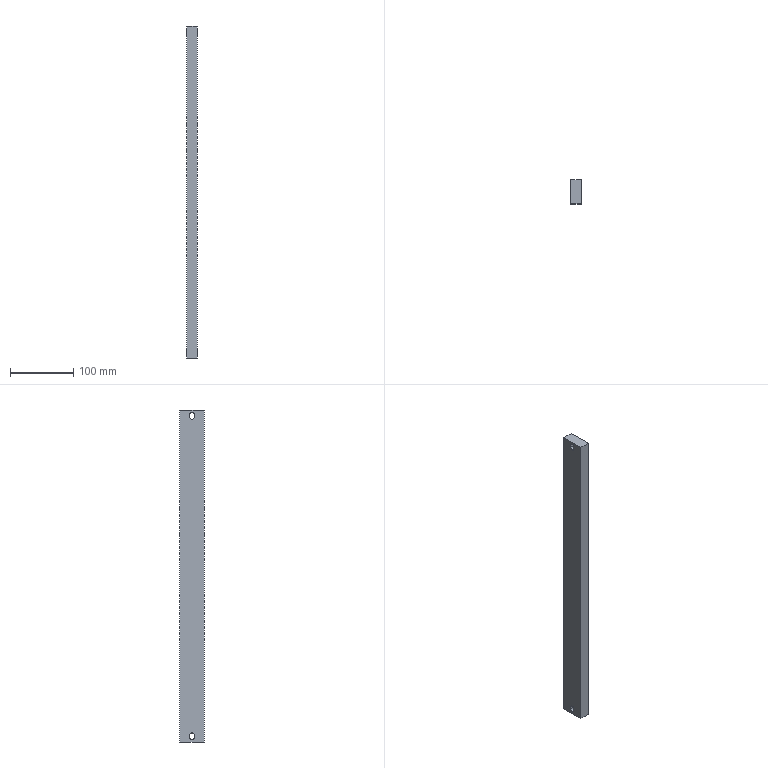Component | SolidWorks | NameDuplicate-1Crossbar-1 | 1 solid | 16 faces | box 16 x 38 x 523 mm | volume 315856 mm3 | plane 10 | cylinder 6 | commonest cylinder face diameters 7 x6
build123d program:
from build123d import *

# Parameters (mm, degrees)
SKETCH1_W           = 523
SKETCH1_H           = 38
BOSS_EXTRUDE1_DEPTH = 16


with BuildPart() as part:
    # Sketch1 → Boss-Extrude1 (new body)
    with BuildSketch(Plane.XY.offset(8)):
        Rectangle(SKETCH1_W, SKETCH1_H)
        with BuildLine():
            Line((-250.5, -3.5), (-254.5, -3.5))
            ThreePointArc((-254.5, -3.5), (-258, 0), (-254.5, 3.5))
            Line((-254.5, 3.5), (-250.5, 3.5))
            ThreePointArc((-250.5, 3.5), (-247, 0), (-250.5, -3.5))
        make_face(mode=Mode.SUBTRACT)
        with BuildLine():
            Line((254.5, -3.5), (250.5, -3.5))
            ThreePointArc((250.5, -3.5), (247, 0), (250.5, 3.5))
            Line((250.5, 3.5), (254.5, 3.5))
            ThreePointArc((254.5, 3.5), (258, 0), (254.5, -3.5))
        make_face(mode=Mode.SUBTRACT)
    extrude(amount=-BOSS_EXTRUDE1_DEPTH)


solid = part.part

# Placed as in the assembly
solid = solid.moved(Location((-405, 406, 0), (0, 90, 0)))
STEP:
#1=CARTESIAN_POINT('',(-15.63,15.984,10.157));
#2=VERTEX_POINT('',#1);
#3=CARTESIAN_POINT('',(-15.63,16.122,10.02));
#4=VERTEX_POINT('',#3);
#5=CARTESIAN_POINT('',(-15.63,15.984,10.02));
#6=DIRECTION('',(-1.,0.,0.));
#7=DIRECTION('',(0.,0.,-1.));
#8=AXIS2_PLACEMENT_3D('',#5,#6,#7);
#9=CIRCLE('',#8,0.1378);
#10=EDGE_CURVE('',#2,#4,#9,.T.);
#11=ORIENTED_EDGE('',*,*,#10,.F.);
#12=CARTESIAN_POINT('',(-16.26,15.984,10.157));
#13=VERTEX_POINT('',#12);
#14=CARTESIAN_POINT('',(-15.63,15.984,10.157));
#15=DIRECTION('',(-1.,0.,0.));
#16=VECTOR('',#15,39.37);
#17=LINE('',#14,#16);
#18=EDGE_CURVE('',#2,#13,#17,.T.);
#19=ORIENTED_EDGE('',*,*,#18,.T.);
#20=CARTESIAN_POINT('',(-16.26,16.122,10.02));
#21=VERTEX_POINT('',#20);
#22=CARTESIAN_POINT('',(-16.26,15.984,10.02));
#23=DIRECTION('',(-1.,0.,0.));
#24=DIRECTION('',(0.,0.,-1.));
#25=AXIS2_PLACEMENT_3D('',#22,#23,#24);
#26=CIRCLE('',#25,0.1378);
#27=EDGE_CURVE('',#13,#21,#26,.T.);
#28=ORIENTED_EDGE('',*,*,#27,.T.);
#29=CARTESIAN_POINT('',(-15.63,16.122,10.02));
#30=DIRECTION('',(-1.,0.,0.));
#31=VECTOR('',#30,39.37);
#32=LINE('',#29,#31);
#33=EDGE_CURVE('',#4,#21,#32,.T.);
#34=ORIENTED_EDGE('',*,*,#33,.F.);
#35=EDGE_LOOP('',(#11,#19,#28,#34));
#36=FACE_OUTER_BOUND('',#35,.T.);
#37=CARTESIAN_POINT('',(-15.63,15.984,10.02));
#38=DIRECTION('',(-1.,0.,0.));
#39=DIRECTION('',(0.,0.,1.));
#40=AXIS2_PLACEMENT_3D('',#37,#38,#39);
#41=CYLINDRICAL_SURFACE('',#40,0.1378);
#42=ADVANCED_FACE('',(#36),#41,.F.);
#43=CARTESIAN_POINT('',(-15.63,15.984,-9.724));
#44=VERTEX_POINT('',#43);
#45=CARTESIAN_POINT('',(-15.63,16.122,-9.862));
#46=VERTEX_POINT('',#45);
#47=CARTESIAN_POINT('',(-15.63,15.984,-9.862));
#48=DIRECTION('',(-1.,0.,0.));
#49=DIRECTION('',(0.,0.,-1.));
#50=AXIS2_PLACEMENT_3D('',#47,#48,#49);
#51=CIRCLE('',#50,0.1378);
#52=EDGE_CURVE('',#44,#46,#51,.T.);
#53=ORIENTED_EDGE('',*,*,#52,.F.);
#54=CARTESIAN_POINT('',(-16.26,15.984,-9.724));
#55=VERTEX_POINT('',#54);
#56=CARTESIAN_POINT('',(-15.63,15.984,-9.724));
#57=DIRECTION('',(-1.,0.,0.));
#58=VECTOR('',#57,39.37);
#59=LINE('',#56,#58);
#60=EDGE_CURVE('',#44,#55,#59,.T.);
#61=ORIENTED_EDGE('',*,*,#60,.T.);
#62=CARTESIAN_POINT('',(-16.26,16.122,-9.862));
#63=VERTEX_POINT('',#62);
#64=CARTESIAN_POINT('',(-16.26,15.984,-9.862));
#65=DIRECTION('',(-1.,0.,0.));
#66=DIRECTION('',(0.,0.,-1.));
#67=AXIS2_PLACEMENT_3D('',#64,#65,#66);
#68=CIRCLE('',#67,0.1378);
#69=EDGE_CURVE('',#55,#63,#68,.T.);
#70=ORIENTED_EDGE('',*,*,#69,.T.);
#71=CARTESIAN_POINT('',(-15.63,16.122,-9.862));
#72=DIRECTION('',(-1.,0.,0.));
#73=VECTOR('',#72,39.37);
#74=LINE('',#71,#73);
#75=EDGE_CURVE('',#46,#63,#74,.T.);
#76=ORIENTED_EDGE('',*,*,#75,.F.);
#77=EDGE_LOOP('',(#53,#61,#70,#76));
#78=FACE_OUTER_BOUND('',#77,.T.);
#79=CARTESIAN_POINT('',(-15.63,15.984,-9.862));
#80=DIRECTION('',(-1.,0.,0.));
#81=DIRECTION('',(0.,0.,1.));
#82=AXIS2_PLACEMENT_3D('',#79,#80,#81);
#83=CYLINDRICAL_SURFACE('',#82,0.1378);
#84=ADVANCED_FACE('',(#78),#83,.F.);
#85=CARTESIAN_POINT('',(-16.26,15.236,-10.295));
#86=VERTEX_POINT('',#85);
#87=CARTESIAN_POINT('',(-16.26,15.236,10.295));
#88=VERTEX_POINT('',#87);
#89=CARTESIAN_POINT('',(-16.26,15.236,-10.295));
#90=DIRECTION('',(0.,0.,1.));
#91=VECTOR('',#90,39.37);
#92=LINE('',#89,#91);
#93=EDGE_CURVE('',#86,#88,#92,.T.);
#94=ORIENTED_EDGE('',*,*,#93,.F.);
#95=CARTESIAN_POINT('',(-15.63,15.236,-10.295));
#96=VERTEX_POINT('',#95);
#97=CARTESIAN_POINT('',(-15.63,15.236,-10.295));
#98=DIRECTION('',(-1.,0.,0.));
#99=VECTOR('',#98,39.37);
#100=LINE('',#97,#99);
#101=EDGE_CURVE('',#96,#86,#100,.T.);
#102=ORIENTED_EDGE('',*,*,#101,.F.);
#103=CARTESIAN_POINT('',(-15.63,15.236,10.295));
#104=VERTEX_POINT('',#103);
#105=CARTESIAN_POINT('',(-15.63,15.236,-10.295));
#106=DIRECTION('',(0.,0.,1.));
#107=VECTOR('',#106,39.37);
#108=LINE('',#105,#107);
#109=EDGE_CURVE('',#96,#104,#108,.T.);
#110=ORIENTED_EDGE('',*,*,#109,.T.);
#111=CARTESIAN_POINT('',(-15.63,15.236,10.295));
#112=DIRECTION('',(-1.,0.,0.));
#113=VECTOR('',#112,39.37);
#114=LINE('',#111,#113);
#115=EDGE_CURVE('',#104,#88,#114,.T.);
#116=ORIENTED_EDGE('',*,*,#115,.T.);
#117=EDGE_LOOP('',(#94,#102,#110,#116));
#118=FACE_OUTER_BOUND('',#117,.T.);
#119=CARTESIAN_POINT('',(-15.63,15.236,-10.295));
#120=DIRECTION('',(-0.,-1.,0.));
#121=DIRECTION('',(1.,-0.,-0.));
#122=AXIS2_PLACEMENT_3D('',#119,#120,#121);
#123=PLANE('',#122);
#124=ADVANCED_FACE('',(#118),#123,.T.);
#125=CARTESIAN_POINT('',(-16.26,16.732,-10.295));
#126=VERTEX_POINT('',#125);
#127=CARTESIAN_POINT('',(-16.26,16.732,-10.295));
#128=DIRECTION('',(-0.,-1.,0.));
#129=VECTOR('',#128,39.37);
#130=LINE('',#127,#129);
#131=EDGE_CURVE('',#126,#86,#130,.T.);
#132=ORIENTED_EDGE('',*,*,#131,.F.);
#133=CARTESIAN_POINT('',(-15.63,16.732,-10.295));
#134=VERTEX_POINT('',#133);
#135=CARTESIAN_POINT('',(-15.63,16.732,-10.295));
#136=DIRECTION('',(-1.,0.,0.));
#137=VECTOR('',#136,39.37);
#138=LINE('',#135,#137);
#139=EDGE_CURVE('',#134,#126,#138,.T.);
#140=ORIENTED_EDGE('',*,*,#139,.F.);
#141=CARTESIAN_POINT('',(-15.63,16.732,-10.295));
#142=DIRECTION('',(-0.,-1.,0.));
#143=VECTOR('',#142,39.37);
#144=LINE('',#141,#143);
#145=EDGE_CURVE('',#134,#96,#144,.T.);
#146=ORIENTED_EDGE('',*,*,#145,.T.);
#147=ORIENTED_EDGE('',*,*,#101,.T.);
#148=EDGE_LOOP('',(#132,#140,#146,#147));
#149=FACE_OUTER_BOUND('',#148,.T.);
#150=CARTESIAN_POINT('',(-15.63,16.732,-10.295));
#151=DIRECTION('',(-0.,-0.,-1.));
#152=DIRECTION('',(-1.,0.,0.));
#153=AXIS2_PLACEMENT_3D('',#150,#151,#152);
#154=PLANE('',#153);
#155=ADVANCED_FACE('',(#149),#154,.T.);
#156=CARTESIAN_POINT('',(-16.26,16.732,10.295));
#157=VERTEX_POINT('',#156);
#158=CARTESIAN_POINT('',(-16.26,16.732,10.295));
#159=DIRECTION('',(-0.,-0.,-1.));
#160=VECTOR('',#159,39.37);
#161=LINE('',#158,#160);
#162=EDGE_CURVE('',#157,#126,#161,.T.);
#163=ORIENTED_EDGE('',*,*,#162,.F.);
#164=CARTESIAN_POINT('',(-15.63,16.732,10.295));
#165=VERTEX_POINT('',#164);
#166=CARTESIAN_POINT('',(-15.63,16.732,10.295));
#167=DIRECTION('',(-1.,0.,0.));
#168=VECTOR('',#167,39.37);
#169=LINE('',#166,#168);
#170=EDGE_CURVE('',#165,#157,#169,.T.);
#171=ORIENTED_EDGE('',*,*,#170,.F.);
#172=CARTESIAN_POINT('',(-15.63,16.732,10.295));
#173=DIRECTION('',(-0.,-0.,-1.));
#174=VECTOR('',#173,39.37);
#175=LINE('',#172,#174);
#176=EDGE_CURVE('',#165,#134,#175,.T.);
#177=ORIENTED_EDGE('',*,*,#176,.T.);
#178=ORIENTED_EDGE('',*,*,#139,.T.);
#179=EDGE_LOOP('',(#163,#171,#177,#178));
#180=FACE_OUTER_BOUND('',#179,.T.);
#181=CARTESIAN_POINT('',(-15.63,16.732,10.295));
#182=DIRECTION('',(0.,1.,-0.));
#183=DIRECTION('',(-0.,-0.,-1.));
#184=AXIS2_PLACEMENT_3D('',#181,#182,#183);
#185=PLANE('',#184);
#186=ADVANCED_FACE('',(#180),#185,.T.);
#187=CARTESIAN_POINT('',(-16.26,15.236,10.295));
#188=DIRECTION('',(0.,1.,-0.));
#189=VECTOR('',#188,39.37);
#190=LINE('',#187,#189);
#191=EDGE_CURVE('',#88,#157,#190,.T.);
#192=ORIENTED_EDGE('',*,*,#191,.F.);
#193=ORIENTED_EDGE('',*,*,#115,.F.);
#194=CARTESIAN_POINT('',(-15.63,15.236,10.295));
#195=DIRECTION('',(0.,1.,-0.));
#196=VECTOR('',#195,39.37);
#197=LINE('',#194,#196);
#198=EDGE_CURVE('',#104,#165,#197,.T.);
#199=ORIENTED_EDGE('',*,*,#198,.T.);
#200=ORIENTED_EDGE('',*,*,#170,.T.);
#201=EDGE_LOOP('',(#192,#193,#199,#200));
#202=FACE_OUTER_BOUND('',#201,.T.);
#203=CARTESIAN_POINT('',(-15.63,15.236,10.295));
#204=DIRECTION('',(0.,0.,1.));
#205=DIRECTION('',(1.,-0.,-0.));
#206=AXIS2_PLACEMENT_3D('',#203,#204,#205);
#207=PLANE('',#206);
#208=ADVANCED_FACE('',(#202),#207,.T.);
#209=CARTESIAN_POINT('',(-15.63,15.846,9.862));
#210=VERTEX_POINT('',#209);
#211=CARTESIAN_POINT('',(-15.63,15.846,10.02));
#212=VERTEX_POINT('',#211);
#213=CARTESIAN_POINT('',(-15.63,15.846,10.02));
#214=DIRECTION('',(0.,0.,1.));
#215=VECTOR('',#214,39.37);
#216=LINE('',#213,#215);
#217=EDGE_CURVE('',#210,#212,#216,.T.);
#218=ORIENTED_EDGE('',*,*,#217,.T.);
#219=CARTESIAN_POINT('',(-15.63,15.984,10.02));
#220=DIRECTION('',(-1.,0.,0.));
#221=DIRECTION('',(0.,0.,-1.));
#222=AXIS2_PLACEMENT_3D('',#219,#220,#221);
#223=CIRCLE('',#222,0.1378);
#224=EDGE_CURVE('',#212,#2,#223,.T.);
#225=ORIENTED_EDGE('',*,*,#224,.T.);
#226=ORIENTED_EDGE('',*,*,#10,.T.);
#227=CARTESIAN_POINT('',(-15.63,16.122,9.862));
#228=VERTEX_POINT('',#227);
#229=CARTESIAN_POINT('',(-15.63,16.122,9.862));
#230=DIRECTION('',(-0.,-0.,-1.));
#231=VECTOR('',#230,39.37);
#232=LINE('',#229,#231);
#233=EDGE_CURVE('',#4,#228,#232,.T.);
#234=ORIENTED_EDGE('',*,*,#233,.T.);
#235=CARTESIAN_POINT('',(-15.63,15.984,9.862));
#236=DIRECTION('',(-1.,0.,0.));
#237=DIRECTION('',(0.,0.,-1.));
#238=AXIS2_PLACEMENT_3D('',#235,#236,#237);
#239=CIRCLE('',#238,0.1378);
#240=EDGE_CURVE('',#228,#210,#239,.T.);
#241=ORIENTED_EDGE('',*,*,#240,.T.);
#242=EDGE_LOOP('',(#218,#225,#226,#234,#241));
#243=FACE_BOUND('',#242,.T.);
#244=CARTESIAN_POINT('',(-15.63,15.846,-10.02));
#245=VERTEX_POINT('',#244);
#246=CARTESIAN_POINT('',(-15.63,15.846,-9.862));
#247=VERTEX_POINT('',#246);
#248=CARTESIAN_POINT('',(-15.63,15.846,-9.862));
#249=DIRECTION('',(0.,0.,1.));
#250=VECTOR('',#249,39.37);
#251=LINE('',#248,#250);
#252=EDGE_CURVE('',#245,#247,#251,.T.);
#253=ORIENTED_EDGE('',*,*,#252,.T.);
#254=CARTESIAN_POINT('',(-15.63,15.984,-9.862));
#255=DIRECTION('',(-1.,0.,0.));
#256=DIRECTION('',(0.,0.,-1.));
#257=AXIS2_PLACEMENT_3D('',#254,#255,#256);
#258=CIRCLE('',#257,0.1378);
#259=EDGE_CURVE('',#247,#44,#258,.T.);
#260=ORIENTED_EDGE('',*,*,#259,.T.);
#261=ORIENTED_EDGE('',*,*,#52,.T.);
#262=CARTESIAN_POINT('',(-15.63,16.122,-10.02));
#263=VERTEX_POINT('',#262);
#264=CARTESIAN_POINT('',(-15.63,16.122,-10.02));
#265=DIRECTION('',(-0.,-0.,-1.));
#266=VECTOR('',#265,39.37);
#267=LINE('',#264,#266);
#268=EDGE_CURVE('',#46,#263,#267,.T.);
#269=ORIENTED_EDGE('',*,*,#268,.T.);
#270=CARTESIAN_POINT('',(-15.63,15.984,-10.02));
#271=DIRECTION('',(-1.,0.,0.));
#272=DIRECTION('',(0.,0.,-1.));
#273=AXIS2_PLACEMENT_3D('',#270,#271,#272);
#274=CIRCLE('',#273,0.1378);
#275=EDGE_CURVE('',#263,#245,#274,.T.);
#276=ORIENTED_EDGE('',*,*,#275,.T.);
#277=EDGE_LOOP('',(#253,#260,#261,#269,#276));
#278=FACE_BOUND('',#277,.T.);
#279=ORIENTED_EDGE('',*,*,#109,.F.);
#280=ORIENTED_EDGE('',*,*,#145,.F.);
#281=ORIENTED_EDGE('',*,*,#176,.F.);
#282=ORIENTED_EDGE('',*,*,#198,.F.);
#283=EDGE_LOOP('',(#279,#280,#281,#282));
#284=FACE_OUTER_BOUND('',#283,.T.);
#285=CARTESIAN_POINT('',(-15.63,15.984,-0.));
#286=DIRECTION('',(-1.,0.,0.));
#287=DIRECTION('',(0.,0.,1.));
#288=AXIS2_PLACEMENT_3D('',#285,#286,#287);
#289=PLANE('',#288);
#290=ADVANCED_FACE('',(#243,#278,#284),#289,.F.);
#291=CARTESIAN_POINT('',(-16.26,15.846,10.02));
#292=VERTEX_POINT('',#291);
#293=CARTESIAN_POINT('',(-16.26,15.984,10.02));
#294=DIRECTION('',(-1.,0.,0.));
#295=DIRECTION('',(0.,0.,-1.));
#296=AXIS2_PLACEMENT_3D('',#293,#294,#295);
#297=CIRCLE('',#296,0.1378);
#298=EDGE_CURVE('',#292,#13,#297,.T.);
#299=ORIENTED_EDGE('',*,*,#298,.F.);
#300=CARTESIAN_POINT('',(-16.26,15.846,9.862));
#301=VERTEX_POINT('',#300);
#302=CARTESIAN_POINT('',(-16.26,15.846,10.02));
#303=DIRECTION('',(0.,0.,1.));
#304=VECTOR('',#303,39.37);
#305=LINE('',#302,#304);
#306=EDGE_CURVE('',#301,#292,#305,.T.);
#307=ORIENTED_EDGE('',*,*,#306,.F.);
#308=CARTESIAN_POINT('',(-16.26,16.122,9.862));
#309=VERTEX_POINT('',#308);
#310=CARTESIAN_POINT('',(-16.26,15.984,9.862));
#311=DIRECTION('',(-1.,0.,0.));
#312=DIRECTION('',(0.,0.,-1.));
#313=AXIS2_PLACEMENT_3D('',#310,#311,#312);
#314=CIRCLE('',#313,0.1378);
#315=EDGE_CURVE('',#309,#301,#314,.T.);
#316=ORIENTED_EDGE('',*,*,#315,.F.);
#317=CARTESIAN_POINT('',(-16.26,16.122,9.862));
#318=DIRECTION('',(-0.,-0.,-1.));
#319=VECTOR('',#318,39.37);
#320=LINE('',#317,#319);
#321=EDGE_CURVE('',#21,#309,#320,.T.);
#322=ORIENTED_EDGE('',*,*,#321,.F.);
#323=ORIENTED_EDGE('',*,*,#27,.F.);
#324=EDGE_LOOP('',(#299,#307,#316,#322,#323));
#325=FACE_BOUND('',#324,.T.);
#326=CARTESIAN_POINT('',(-16.26,15.846,-9.862));
#327=VERTEX_POINT('',#326);
#328=CARTESIAN_POINT('',(-16.26,15.984,-9.862));
#329=DIRECTION('',(-1.,0.,0.));
#330=DIRECTION('',(0.,0.,-1.));
#331=AXIS2_PLACEMENT_3D('',#328,#329,#330);
#332=CIRCLE('',#331,0.1378);
#333=EDGE_CURVE('',#327,#55,#332,.T.);
#334=ORIENTED_EDGE('',*,*,#333,.F.);
#335=CARTESIAN_POINT('',(-16.26,15.846,-10.02));
#336=VERTEX_POINT('',#335);
#337=CARTESIAN_POINT('',(-16.26,15.846,-9.862));
#338=DIRECTION('',(0.,0.,1.));
#339=VECTOR('',#338,39.37);
#340=LINE('',#337,#339);
#341=EDGE_CURVE('',#336,#327,#340,.T.);
#342=ORIENTED_EDGE('',*,*,#341,.F.);
#343=CARTESIAN_POINT('',(-16.26,16.122,-10.02));
#344=VERTEX_POINT('',#343);
#345=CARTESIAN_POINT('',(-16.26,15.984,-10.02));
#346=DIRECTION('',(-1.,0.,0.));
#347=DIRECTION('',(0.,0.,-1.));
#348=AXIS2_PLACEMENT_3D('',#345,#346,#347);
#349=CIRCLE('',#348,0.1378);
#350=EDGE_CURVE('',#344,#336,#349,.T.);
#351=ORIENTED_EDGE('',*,*,#350,.F.);
#352=CARTESIAN_POINT('',(-16.26,16.122,-10.02));
#353=DIRECTION('',(-0.,-0.,-1.));
#354=VECTOR('',#353,39.37);
#355=LINE('',#352,#354);
#356=EDGE_CURVE('',#63,#344,#355,.T.);
#357=ORIENTED_EDGE('',*,*,#356,.F.);
#358=ORIENTED_EDGE('',*,*,#69,.F.);
#359=EDGE_LOOP('',(#334,#342,#351,#357,#358));
#360=FACE_BOUND('',#359,.T.);
#361=ORIENTED_EDGE('',*,*,#93,.T.);
#362=ORIENTED_EDGE('',*,*,#191,.T.);
#363=ORIENTED_EDGE('',*,*,#162,.T.);
#364=ORIENTED_EDGE('',*,*,#131,.T.);
#365=EDGE_LOOP('',(#361,#362,#363,#364));
#366=FACE_OUTER_BOUND('',#365,.T.);
#367=CARTESIAN_POINT('',(-16.26,15.984,-0.));
#368=DIRECTION('',(-1.,0.,0.));
#369=DIRECTION('',(0.,0.,1.));
#370=AXIS2_PLACEMENT_3D('',#367,#368,#369);
#371=PLANE('',#370);
#372=ADVANCED_FACE('',(#325,#360,#366),#371,.T.);
#373=ORIENTED_EDGE('',*,*,#60,.F.);
#374=ORIENTED_EDGE('',*,*,#259,.F.);
#375=CARTESIAN_POINT('',(-15.63,15.846,-9.862));
#376=DIRECTION('',(-1.,0.,0.));
#377=VECTOR('',#376,39.37);
#378=LINE('',#375,#377);
#379=EDGE_CURVE('',#247,#327,#378,.T.);
#380=ORIENTED_EDGE('',*,*,#379,.T.);
#381=ORIENTED_EDGE('',*,*,#333,.T.);
#382=EDGE_LOOP('',(#373,#374,#380,#381));
#383=FACE_OUTER_BOUND('',#382,.T.);
#384=CARTESIAN_POINT('',(-15.63,15.984,-9.862));
#385=DIRECTION('',(-1.,0.,0.));
#386=DIRECTION('',(0.,0.,1.));
#387=AXIS2_PLACEMENT_3D('',#384,#385,#386);
#388=CYLINDRICAL_SURFACE('',#387,0.1378);
#389=ADVANCED_FACE('',(#383),#388,.F.);
#390=ORIENTED_EDGE('',*,*,#341,.T.);
#391=ORIENTED_EDGE('',*,*,#379,.F.);
#392=ORIENTED_EDGE('',*,*,#252,.F.);
#393=CARTESIAN_POINT('',(-15.63,15.846,-10.02));
#394=DIRECTION('',(-1.,0.,0.));
#395=VECTOR('',#394,39.37);
#396=LINE('',#393,#395);
#397=EDGE_CURVE('',#245,#336,#396,.T.);
#398=ORIENTED_EDGE('',*,*,#397,.T.);
#399=EDGE_LOOP('',(#390,#391,#392,#398));
#400=FACE_OUTER_BOUND('',#399,.T.);
#401=CARTESIAN_POINT('',(-15.63,15.846,-9.862));
#402=DIRECTION('',(-0.,-1.,0.));
#403=DIRECTION('',(0.,0.,1.));
#404=AXIS2_PLACEMENT_3D('',#401,#402,#403);
#405=PLANE('',#404);
#406=ADVANCED_FACE('',(#400),#405,.F.);
#407=ORIENTED_EDGE('',*,*,#350,.T.);
#408=ORIENTED_EDGE('',*,*,#397,.F.);
#409=ORIENTED_EDGE('',*,*,#275,.F.);
#410=CARTESIAN_POINT('',(-15.63,16.122,-10.02));
#411=DIRECTION('',(-1.,0.,0.));
#412=VECTOR('',#411,39.37);
#413=LINE('',#410,#412);
#414=EDGE_CURVE('',#263,#344,#413,.T.);
#415=ORIENTED_EDGE('',*,*,#414,.T.);
#416=EDGE_LOOP('',(#407,#408,#409,#415));
#417=FACE_OUTER_BOUND('',#416,.T.);
#418=CARTESIAN_POINT('',(-15.63,15.984,-10.02));
#419=DIRECTION('',(-1.,0.,0.));
#420=DIRECTION('',(0.,0.,1.));
#421=AXIS2_PLACEMENT_3D('',#418,#419,#420);
#422=CYLINDRICAL_SURFACE('',#421,0.1378);
#423=ADVANCED_FACE('',(#417),#422,.F.);
#424=ORIENTED_EDGE('',*,*,#356,.T.);
#425=ORIENTED_EDGE('',*,*,#414,.F.);
#426=ORIENTED_EDGE('',*,*,#268,.F.);
#427=ORIENTED_EDGE('',*,*,#75,.T.);
#428=EDGE_LOOP('',(#424,#425,#426,#427));
#429=FACE_OUTER_BOUND('',#428,.T.);
#430=CARTESIAN_POINT('',(-15.63,16.122,-10.02));
#431=DIRECTION('',(0.,1.,-0.));
#432=DIRECTION('',(-0.,-0.,-1.));
#433=AXIS2_PLACEMENT_3D('',#430,#431,#432);
#434=PLANE('',#433);
#435=ADVANCED_FACE('',(#429),#434,.F.);
#436=ORIENTED_EDGE('',*,*,#18,.F.);
#437=ORIENTED_EDGE('',*,*,#224,.F.);
#438=CARTESIAN_POINT('',(-15.63,15.846,10.02));
#439=DIRECTION('',(-1.,0.,0.));
#440=VECTOR('',#439,39.37);
#441=LINE('',#438,#440);
#442=EDGE_CURVE('',#212,#292,#441,.T.);
#443=ORIENTED_EDGE('',*,*,#442,.T.);
#444=ORIENTED_EDGE('',*,*,#298,.T.);
#445=EDGE_LOOP('',(#436,#437,#443,#444));
#446=FACE_OUTER_BOUND('',#445,.T.);
#447=CARTESIAN_POINT('',(-15.63,15.984,10.02));
#448=DIRECTION('',(-1.,0.,0.));
#449=DIRECTION('',(0.,0.,1.));
#450=AXIS2_PLACEMENT_3D('',#447,#448,#449);
#451=CYLINDRICAL_SURFACE('',#450,0.1378);
#452=ADVANCED_FACE('',(#446),#451,.F.);
#453=ORIENTED_EDGE('',*,*,#306,.T.);
#454=ORIENTED_EDGE('',*,*,#442,.F.);
#455=ORIENTED_EDGE('',*,*,#217,.F.);
#456=CARTESIAN_POINT('',(-15.63,15.846,9.862));
#457=DIRECTION('',(-1.,0.,0.));
#458=VECTOR('',#457,39.37);
#459=LINE('',#456,#458);
#460=EDGE_CURVE('',#210,#301,#459,.T.);
#461=ORIENTED_EDGE('',*,*,#460,.T.);
#462=EDGE_LOOP('',(#453,#454,#455,#461));
#463=FACE_OUTER_BOUND('',#462,.T.);
#464=CARTESIAN_POINT('',(-15.63,15.846,10.02));
#465=DIRECTION('',(-0.,-1.,0.));
#466=DIRECTION('',(0.,0.,1.));
#467=AXIS2_PLACEMENT_3D('',#464,#465,#466);
#468=PLANE('',#467);
#469=ADVANCED_FACE('',(#463),#468,.F.);
#470=ORIENTED_EDGE('',*,*,#315,.T.);
#471=ORIENTED_EDGE('',*,*,#460,.F.);
#472=ORIENTED_EDGE('',*,*,#240,.F.);
#473=CARTESIAN_POINT('',(-15.63,16.122,9.862));
#474=DIRECTION('',(-1.,0.,0.));
#475=VECTOR('',#474,39.37);
#476=LINE('',#473,#475);
#477=EDGE_CURVE('',#228,#309,#476,.T.);
#478=ORIENTED_EDGE('',*,*,#477,.T.);
#479=EDGE_LOOP('',(#470,#471,#472,#478));
#480=FACE_OUTER_BOUND('',#479,.T.);
#481=CARTESIAN_POINT('',(-15.63,15.984,9.862));
#482=DIRECTION('',(-1.,0.,0.));
#483=DIRECTION('',(0.,0.,1.));
#484=AXIS2_PLACEMENT_3D('',#481,#482,#483);
#485=CYLINDRICAL_SURFACE('',#484,0.1378);
#486=ADVANCED_FACE('',(#480),#485,.F.);
#487=ORIENTED_EDGE('',*,*,#321,.T.);
#488=ORIENTED_EDGE('',*,*,#477,.F.);
#489=ORIENTED_EDGE('',*,*,#233,.F.);
#490=ORIENTED_EDGE('',*,*,#33,.T.);
#491=EDGE_LOOP('',(#487,#488,#489,#490));
#492=FACE_OUTER_BOUND('',#491,.T.);
#493=CARTESIAN_POINT('',(-15.63,16.122,9.862));
#494=DIRECTION('',(0.,1.,-0.));
#495=DIRECTION('',(-0.,-0.,-1.));
#496=AXIS2_PLACEMENT_3D('',#493,#494,#495);
#497=PLANE('',#496);
#498=ADVANCED_FACE('',(#492),#497,.F.);
#499=CLOSED_SHELL('',(#42,#84,#124,#155,#186,#208,#290,#372,#389,#406,#423,#435,#452,#469,#486,#498));
#500=MANIFOLD_SOLID_BREP('',#499);
#501=CARTESIAN_POINT('',(0.,0.,0.));
#502=DIRECTION('',(0.,0.,1.));
#503=DIRECTION('',(1.,0.,0.));
#504=AXIS2_PLACEMENT_3D('',#501,#502,#503);
#505=(LENGTH_UNIT()NAMED_UNIT(*)SI_UNIT($,.METRE.));
#506=LENGTH_MEASURE_WITH_UNIT(LENGTH_MEASURE(0.0254),#505);
#507=DIMENSIONAL_EXPONENTS(1.,0.,0.,0.,0.,0.,0.);
#508=(CONVERSION_BASED_UNIT('',#506)LENGTH_UNIT()NAMED_UNIT(#507));
#509=UNCERTAINTY_MEASURE_WITH_UNIT(LENGTH_MEASURE(0.00001),#508,'','');
#510=(NAMED_UNIT(*)PLANE_ANGLE_UNIT()SI_UNIT($,.RADIAN.));
#511=(NAMED_UNIT(*)SI_UNIT($,.STERADIAN.)SOLID_ANGLE_UNIT());
#512=(GEOMETRIC_REPRESENTATION_CONTEXT(3)GLOBAL_UNCERTAINTY_ASSIGNED_CONTEXT((#509))GLOBAL_UNIT_ASSIGNED_CONTEXT((#508,#510,#511))REPRESENTATION_CONTEXT('',''));
#513=ADVANCED_BREP_SHAPE_REPRESENTATION('',(#500,#504),#512);
#514=COLOUR_RGB('',0.7922,0.8196,0.9333);
#515=FILL_AREA_STYLE_COLOUR('',#514);
#516=FILL_AREA_STYLE('',(#515));
#517=SURFACE_STYLE_FILL_AREA(#516);
#518=SURFACE_SIDE_STYLE('',(#517));
#519=SURFACE_STYLE_USAGE(.BOTH.,#518);
#520=PRESENTATION_STYLE_ASSIGNMENT((#519));
#521=STYLED_ITEM('',(#520),#500);
#522=PRESENTATION_LAYER_ASSIGNMENT('','',(#521));
#523=(LENGTH_UNIT()NAMED_UNIT(*)SI_UNIT($,.METRE.));
#524=LENGTH_MEASURE_WITH_UNIT(LENGTH_MEASURE(0.0254),#523);
#525=DIMENSIONAL_EXPONENTS(1.,0.,0.,0.,0.,0.,0.);
#526=(CONVERSION_BASED_UNIT('',#524)LENGTH_UNIT()NAMED_UNIT(#525));
#527=UNCERTAINTY_MEASURE_WITH_UNIT(LENGTH_MEASURE(0.00001),#526,'','');
#528=(NAMED_UNIT(*)PLANE_ANGLE_UNIT()SI_UNIT($,.RADIAN.));
#529=(NAMED_UNIT(*)SI_UNIT($,.STERADIAN.)SOLID_ANGLE_UNIT());
#530=(GEOMETRIC_REPRESENTATION_CONTEXT(3)GLOBAL_UNCERTAINTY_ASSIGNED_CONTEXT((#527))GLOBAL_UNIT_ASSIGNED_CONTEXT((#526,#528,#529))REPRESENTATION_CONTEXT('',''));
#531=MECHANICAL_DESIGN_GEOMETRIC_PRESENTATION_REPRESENTATION('',(#521),#530);